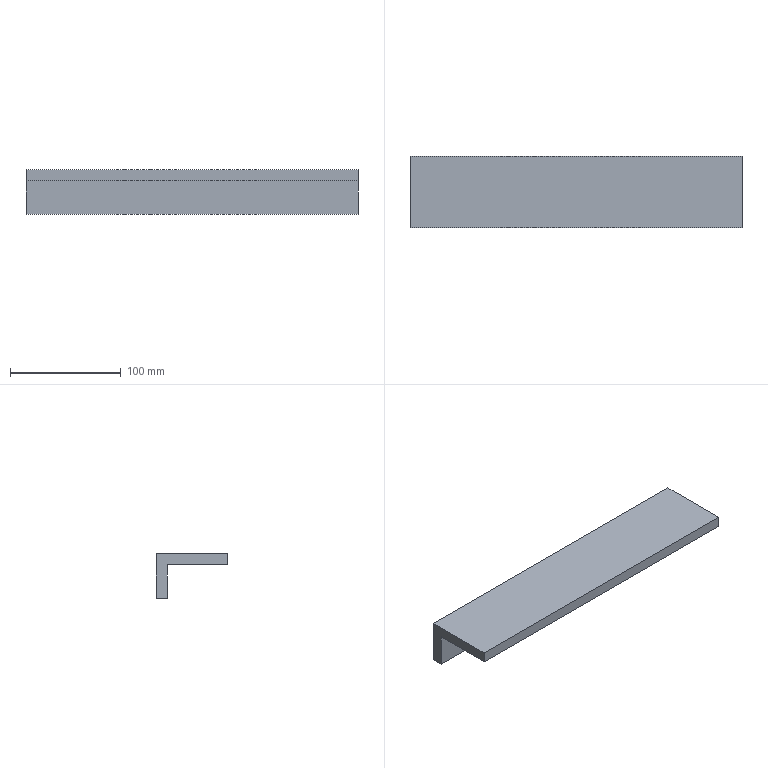Component | SolidWorks | AD12-160328-001K.SDPRT-1 | 1 solid | 8 faces | box 300 x 65 x 40 mm | volume 285000 mm3 | plane 8
build123d program:
from build123d import *

# Parameters (mm, degrees)
BOSS_EXTRUDE1_DEPTH = 150


with BuildPart() as part:
    # Sketch1 → Boss-Extrude1 (new, symmetric)
    with BuildSketch(Plane.XY):
        Polygon((0, 0), (-65, 0), (-65, -40), (-55, -40), (-55, -10), (0, -10), align=None)
    extrude(amount=BOSS_EXTRUDE1_DEPTH, both=True)


solid = part.part

# Placed as in the assembly
solid = solid.moved(Location((-179.414, -253.961, 297.437), (90, -90, 0)))
STEP:
#1=CARTESIAN_POINT('',(-1.158,-9.998,11.316));
#2=VERTEX_POINT('',#1);
#3=CARTESIAN_POINT('',(-1.158,-9.998,11.71));
#4=VERTEX_POINT('',#3);
#5=CARTESIAN_POINT('',(-1.158,-9.998,11.316));
#6=DIRECTION('',(0.,-0.,1.));
#7=VECTOR('',#6,39.37);
#8=LINE('',#5,#7);
#9=EDGE_CURVE('',#2,#4,#8,.T.);
#10=ORIENTED_EDGE('',*,*,#9,.T.);
#11=CARTESIAN_POINT('',(-12.969,-9.998,11.71));
#12=VERTEX_POINT('',#11);
#13=CARTESIAN_POINT('',(-12.969,-9.998,11.71));
#14=DIRECTION('',(1.,-0.,0.));
#15=VECTOR('',#14,39.37);
#16=LINE('',#13,#15);
#17=EDGE_CURVE('',#12,#4,#16,.T.);
#18=ORIENTED_EDGE('',*,*,#17,.F.);
#19=CARTESIAN_POINT('',(-12.969,-9.998,11.316));
#20=VERTEX_POINT('',#19);
#21=CARTESIAN_POINT('',(-12.969,-9.998,11.316));
#22=DIRECTION('',(0.,-0.,1.));
#23=VECTOR('',#22,39.37);
#24=LINE('',#21,#23);
#25=EDGE_CURVE('',#20,#12,#24,.T.);
#26=ORIENTED_EDGE('',*,*,#25,.F.);
#27=CARTESIAN_POINT('',(-12.969,-9.998,11.316));
#28=DIRECTION('',(1.,-0.,0.));
#29=VECTOR('',#28,39.37);
#30=LINE('',#27,#29);
#31=EDGE_CURVE('',#20,#2,#30,.T.);
#32=ORIENTED_EDGE('',*,*,#31,.T.);
#33=EDGE_LOOP('',(#10,#18,#26,#32));
#34=FACE_OUTER_BOUND('',#33,.T.);
#35=CARTESIAN_POINT('',(-12.969,-9.998,11.316));
#36=DIRECTION('',(0.,1.,0.));
#37=DIRECTION('',(-1.,0.,0.));
#38=AXIS2_PLACEMENT_3D('',#35,#36,#37);
#39=PLANE('',#38);
#40=ADVANCED_FACE('',(#34),#39,.F.);
#41=CARTESIAN_POINT('',(-1.158,-7.439,11.71));
#42=VERTEX_POINT('',#41);
#43=CARTESIAN_POINT('',(-1.158,-9.998,11.71));
#44=DIRECTION('',(0.,1.,0.));
#45=VECTOR('',#44,39.37);
#46=LINE('',#43,#45);
#47=EDGE_CURVE('',#4,#42,#46,.T.);
#48=ORIENTED_EDGE('',*,*,#47,.T.);
#49=CARTESIAN_POINT('',(-12.969,-7.439,11.71));
#50=VERTEX_POINT('',#49);
#51=CARTESIAN_POINT('',(-12.969,-7.439,11.71));
#52=DIRECTION('',(1.,-0.,0.));
#53=VECTOR('',#52,39.37);
#54=LINE('',#51,#53);
#55=EDGE_CURVE('',#50,#42,#54,.T.);
#56=ORIENTED_EDGE('',*,*,#55,.F.);
#57=CARTESIAN_POINT('',(-12.969,-9.998,11.71));
#58=DIRECTION('',(0.,1.,0.));
#59=VECTOR('',#58,39.37);
#60=LINE('',#57,#59);
#61=EDGE_CURVE('',#12,#50,#60,.T.);
#62=ORIENTED_EDGE('',*,*,#61,.F.);
#63=ORIENTED_EDGE('',*,*,#17,.T.);
#64=EDGE_LOOP('',(#48,#56,#62,#63));
#65=FACE_OUTER_BOUND('',#64,.T.);
#66=CARTESIAN_POINT('',(-12.969,-9.998,11.71));
#67=DIRECTION('',(0.,0.,-1.));
#68=DIRECTION('',(0.,-1.,-0.));
#69=AXIS2_PLACEMENT_3D('',#66,#67,#68);
#70=PLANE('',#69);
#71=ADVANCED_FACE('',(#65),#70,.F.);
#72=CARTESIAN_POINT('',(-1.158,-7.439,10.135));
#73=VERTEX_POINT('',#72);
#74=CARTESIAN_POINT('',(-1.158,-7.439,11.71));
#75=DIRECTION('',(0.,0.,-1.));
#76=VECTOR('',#75,39.37);
#77=LINE('',#74,#76);
#78=EDGE_CURVE('',#42,#73,#77,.T.);
#79=ORIENTED_EDGE('',*,*,#78,.T.);
#80=CARTESIAN_POINT('',(-12.969,-7.439,10.135));
#81=VERTEX_POINT('',#80);
#82=CARTESIAN_POINT('',(-12.969,-7.439,10.135));
#83=DIRECTION('',(1.,-0.,0.));
#84=VECTOR('',#83,39.37);
#85=LINE('',#82,#84);
#86=EDGE_CURVE('',#81,#73,#85,.T.);
#87=ORIENTED_EDGE('',*,*,#86,.F.);
#88=CARTESIAN_POINT('',(-12.969,-7.439,11.71));
#89=DIRECTION('',(0.,0.,-1.));
#90=VECTOR('',#89,39.37);
#91=LINE('',#88,#90);
#92=EDGE_CURVE('',#50,#81,#91,.T.);
#93=ORIENTED_EDGE('',*,*,#92,.F.);
#94=ORIENTED_EDGE('',*,*,#55,.T.);
#95=EDGE_LOOP('',(#79,#87,#93,#94));
#96=FACE_OUTER_BOUND('',#95,.T.);
#97=CARTESIAN_POINT('',(-12.969,-7.439,11.71));
#98=DIRECTION('',(-0.,-1.,-0.));
#99=DIRECTION('',(1.,-0.,0.));
#100=AXIS2_PLACEMENT_3D('',#97,#98,#99);
#101=PLANE('',#100);
#102=ADVANCED_FACE('',(#96),#101,.F.);
#103=CARTESIAN_POINT('',(-1.158,-7.833,10.135));
#104=VERTEX_POINT('',#103);
#105=CARTESIAN_POINT('',(-1.158,-7.439,10.135));
#106=DIRECTION('',(0.,-1.,-0.));
#107=VECTOR('',#106,39.37);
#108=LINE('',#105,#107);
#109=EDGE_CURVE('',#73,#104,#108,.T.);
#110=ORIENTED_EDGE('',*,*,#109,.T.);
#111=CARTESIAN_POINT('',(-12.969,-7.833,10.135));
#112=VERTEX_POINT('',#111);
#113=CARTESIAN_POINT('',(-12.969,-7.833,10.135));
#114=DIRECTION('',(1.,-0.,0.));
#115=VECTOR('',#114,39.37);
#116=LINE('',#113,#115);
#117=EDGE_CURVE('',#112,#104,#116,.T.);
#118=ORIENTED_EDGE('',*,*,#117,.F.);
#119=CARTESIAN_POINT('',(-12.969,-7.439,10.135));
#120=DIRECTION('',(0.,-1.,-0.));
#121=VECTOR('',#120,39.37);
#122=LINE('',#119,#121);
#123=EDGE_CURVE('',#81,#112,#122,.T.);
#124=ORIENTED_EDGE('',*,*,#123,.F.);
#125=ORIENTED_EDGE('',*,*,#86,.T.);
#126=EDGE_LOOP('',(#110,#118,#124,#125));
#127=FACE_OUTER_BOUND('',#126,.T.);
#128=CARTESIAN_POINT('',(-12.969,-7.439,10.135));
#129=DIRECTION('',(-0.,-0.,1.));
#130=DIRECTION('',(-1.,0.,0.));
#131=AXIS2_PLACEMENT_3D('',#128,#129,#130);
#132=PLANE('',#131);
#133=ADVANCED_FACE('',(#127),#132,.F.);
#134=CARTESIAN_POINT('',(-1.158,-7.833,11.316));
#135=VERTEX_POINT('',#134);
#136=CARTESIAN_POINT('',(-1.158,-7.833,10.135));
#137=DIRECTION('',(0.,-0.,1.));
#138=VECTOR('',#137,39.37);
#139=LINE('',#136,#138);
#140=EDGE_CURVE('',#104,#135,#139,.T.);
#141=ORIENTED_EDGE('',*,*,#140,.T.);
#142=CARTESIAN_POINT('',(-12.969,-7.833,11.316));
#143=VERTEX_POINT('',#142);
#144=CARTESIAN_POINT('',(-12.969,-7.833,11.316));
#145=DIRECTION('',(1.,-0.,0.));
#146=VECTOR('',#145,39.37);
#147=LINE('',#144,#146);
#148=EDGE_CURVE('',#143,#135,#147,.T.);
#149=ORIENTED_EDGE('',*,*,#148,.F.);
#150=CARTESIAN_POINT('',(-12.969,-7.833,10.135));
#151=DIRECTION('',(0.,-0.,1.));
#152=VECTOR('',#151,39.37);
#153=LINE('',#150,#152);
#154=EDGE_CURVE('',#112,#143,#153,.T.);
#155=ORIENTED_EDGE('',*,*,#154,.F.);
#156=ORIENTED_EDGE('',*,*,#117,.T.);
#157=EDGE_LOOP('',(#141,#149,#155,#156));
#158=FACE_OUTER_BOUND('',#157,.T.);
#159=CARTESIAN_POINT('',(-12.969,-7.833,10.135));
#160=DIRECTION('',(0.,1.,0.));
#161=DIRECTION('',(-1.,0.,0.));
#162=AXIS2_PLACEMENT_3D('',#159,#160,#161);
#163=PLANE('',#162);
#164=ADVANCED_FACE('',(#158),#163,.F.);
#165=CARTESIAN_POINT('',(-1.158,-7.833,11.316));
#166=DIRECTION('',(0.,-1.,-0.));
#167=VECTOR('',#166,39.37);
#168=LINE('',#165,#167);
#169=EDGE_CURVE('',#135,#2,#168,.T.);
#170=ORIENTED_EDGE('',*,*,#169,.T.);
#171=ORIENTED_EDGE('',*,*,#31,.F.);
#172=CARTESIAN_POINT('',(-12.969,-7.833,11.316));
#173=DIRECTION('',(0.,-1.,-0.));
#174=VECTOR('',#173,39.37);
#175=LINE('',#172,#174);
#176=EDGE_CURVE('',#143,#20,#175,.T.);
#177=ORIENTED_EDGE('',*,*,#176,.F.);
#178=ORIENTED_EDGE('',*,*,#148,.T.);
#179=EDGE_LOOP('',(#170,#171,#177,#178));
#180=FACE_OUTER_BOUND('',#179,.T.);
#181=CARTESIAN_POINT('',(-12.969,-7.833,11.316));
#182=DIRECTION('',(-0.,-0.,1.));
#183=DIRECTION('',(-1.,0.,0.));
#184=AXIS2_PLACEMENT_3D('',#181,#182,#183);
#185=PLANE('',#184);
#186=ADVANCED_FACE('',(#180),#185,.F.);
#187=ORIENTED_EDGE('',*,*,#25,.T.);
#188=ORIENTED_EDGE('',*,*,#61,.T.);
#189=ORIENTED_EDGE('',*,*,#92,.T.);
#190=ORIENTED_EDGE('',*,*,#123,.T.);
#191=ORIENTED_EDGE('',*,*,#154,.T.);
#192=ORIENTED_EDGE('',*,*,#176,.T.);
#193=EDGE_LOOP('',(#187,#188,#189,#190,#191,#192));
#194=FACE_OUTER_BOUND('',#193,.T.);
#195=CARTESIAN_POINT('',(-12.969,-9.998,11.71));
#196=DIRECTION('',(-1.,0.,-0.));
#197=DIRECTION('',(0.,-1.,-0.));
#198=AXIS2_PLACEMENT_3D('',#195,#196,#197);
#199=PLANE('',#198);
#200=ADVANCED_FACE('',(#194),#199,.T.);
#201=ORIENTED_EDGE('',*,*,#9,.F.);
#202=ORIENTED_EDGE('',*,*,#169,.F.);
#203=ORIENTED_EDGE('',*,*,#140,.F.);
#204=ORIENTED_EDGE('',*,*,#109,.F.);
#205=ORIENTED_EDGE('',*,*,#78,.F.);
#206=ORIENTED_EDGE('',*,*,#47,.F.);
#207=EDGE_LOOP('',(#201,#202,#203,#204,#205,#206));
#208=FACE_OUTER_BOUND('',#207,.T.);
#209=CARTESIAN_POINT('',(-1.158,-9.998,11.71));
#210=DIRECTION('',(-1.,0.,-0.));
#211=DIRECTION('',(0.,-1.,-0.));
#212=AXIS2_PLACEMENT_3D('',#209,#210,#211);
#213=PLANE('',#212);
#214=ADVANCED_FACE('',(#208),#213,.F.);
#215=CLOSED_SHELL('',(#40,#71,#102,#133,#164,#186,#200,#214));
#216=MANIFOLD_SOLID_BREP('',#215);
#217=CARTESIAN_POINT('',(0.,0.,0.));
#218=DIRECTION('',(0.,0.,1.));
#219=DIRECTION('',(1.,0.,0.));
#220=AXIS2_PLACEMENT_3D('',#217,#218,#219);
#221=(LENGTH_UNIT()NAMED_UNIT(*)SI_UNIT($,.METRE.));
#222=LENGTH_MEASURE_WITH_UNIT(LENGTH_MEASURE(0.0254),#221);
#223=DIMENSIONAL_EXPONENTS(1.,0.,0.,0.,0.,0.,0.);
#224=(CONVERSION_BASED_UNIT('',#222)LENGTH_UNIT()NAMED_UNIT(#223));
#225=UNCERTAINTY_MEASURE_WITH_UNIT(LENGTH_MEASURE(0.00001),#224,'','');
#226=(NAMED_UNIT(*)PLANE_ANGLE_UNIT()SI_UNIT($,.RADIAN.));
#227=(NAMED_UNIT(*)SI_UNIT($,.STERADIAN.)SOLID_ANGLE_UNIT());
#228=(GEOMETRIC_REPRESENTATION_CONTEXT(3)GLOBAL_UNCERTAINTY_ASSIGNED_CONTEXT((#225))GLOBAL_UNIT_ASSIGNED_CONTEXT((#224,#226,#227))REPRESENTATION_CONTEXT('',''));
#229=ADVANCED_BREP_SHAPE_REPRESENTATION('',(#216,#220),#228);
#230=COLOUR_RGB('',0.7922,0.8196,0.9333);
#231=FILL_AREA_STYLE_COLOUR('',#230);
#232=FILL_AREA_STYLE('',(#231));
#233=SURFACE_STYLE_FILL_AREA(#232);
#234=SURFACE_SIDE_STYLE('',(#233));
#235=SURFACE_STYLE_USAGE(.BOTH.,#234);
#236=PRESENTATION_STYLE_ASSIGNMENT((#235));
#237=STYLED_ITEM('',(#236),#216);
#238=PRESENTATION_LAYER_ASSIGNMENT('','',(#237));
#239=(LENGTH_UNIT()NAMED_UNIT(*)SI_UNIT($,.METRE.));
#240=LENGTH_MEASURE_WITH_UNIT(LENGTH_MEASURE(0.0254),#239);
#241=DIMENSIONAL_EXPONENTS(1.,0.,0.,0.,0.,0.,0.);
#242=(CONVERSION_BASED_UNIT('',#240)LENGTH_UNIT()NAMED_UNIT(#241));
#243=UNCERTAINTY_MEASURE_WITH_UNIT(LENGTH_MEASURE(0.00001),#242,'','');
#244=(NAMED_UNIT(*)PLANE_ANGLE_UNIT()SI_UNIT($,.RADIAN.));
#245=(NAMED_UNIT(*)SI_UNIT($,.STERADIAN.)SOLID_ANGLE_UNIT());
#246=(GEOMETRIC_REPRESENTATION_CONTEXT(3)GLOBAL_UNCERTAINTY_ASSIGNED_CONTEXT((#243))GLOBAL_UNIT_ASSIGNED_CONTEXT((#242,#244,#245))REPRESENTATION_CONTEXT('',''));
#247=MECHANICAL_DESIGN_GEOMETRIC_PRESENTATION_REPRESENTATION('',(#237),#246);